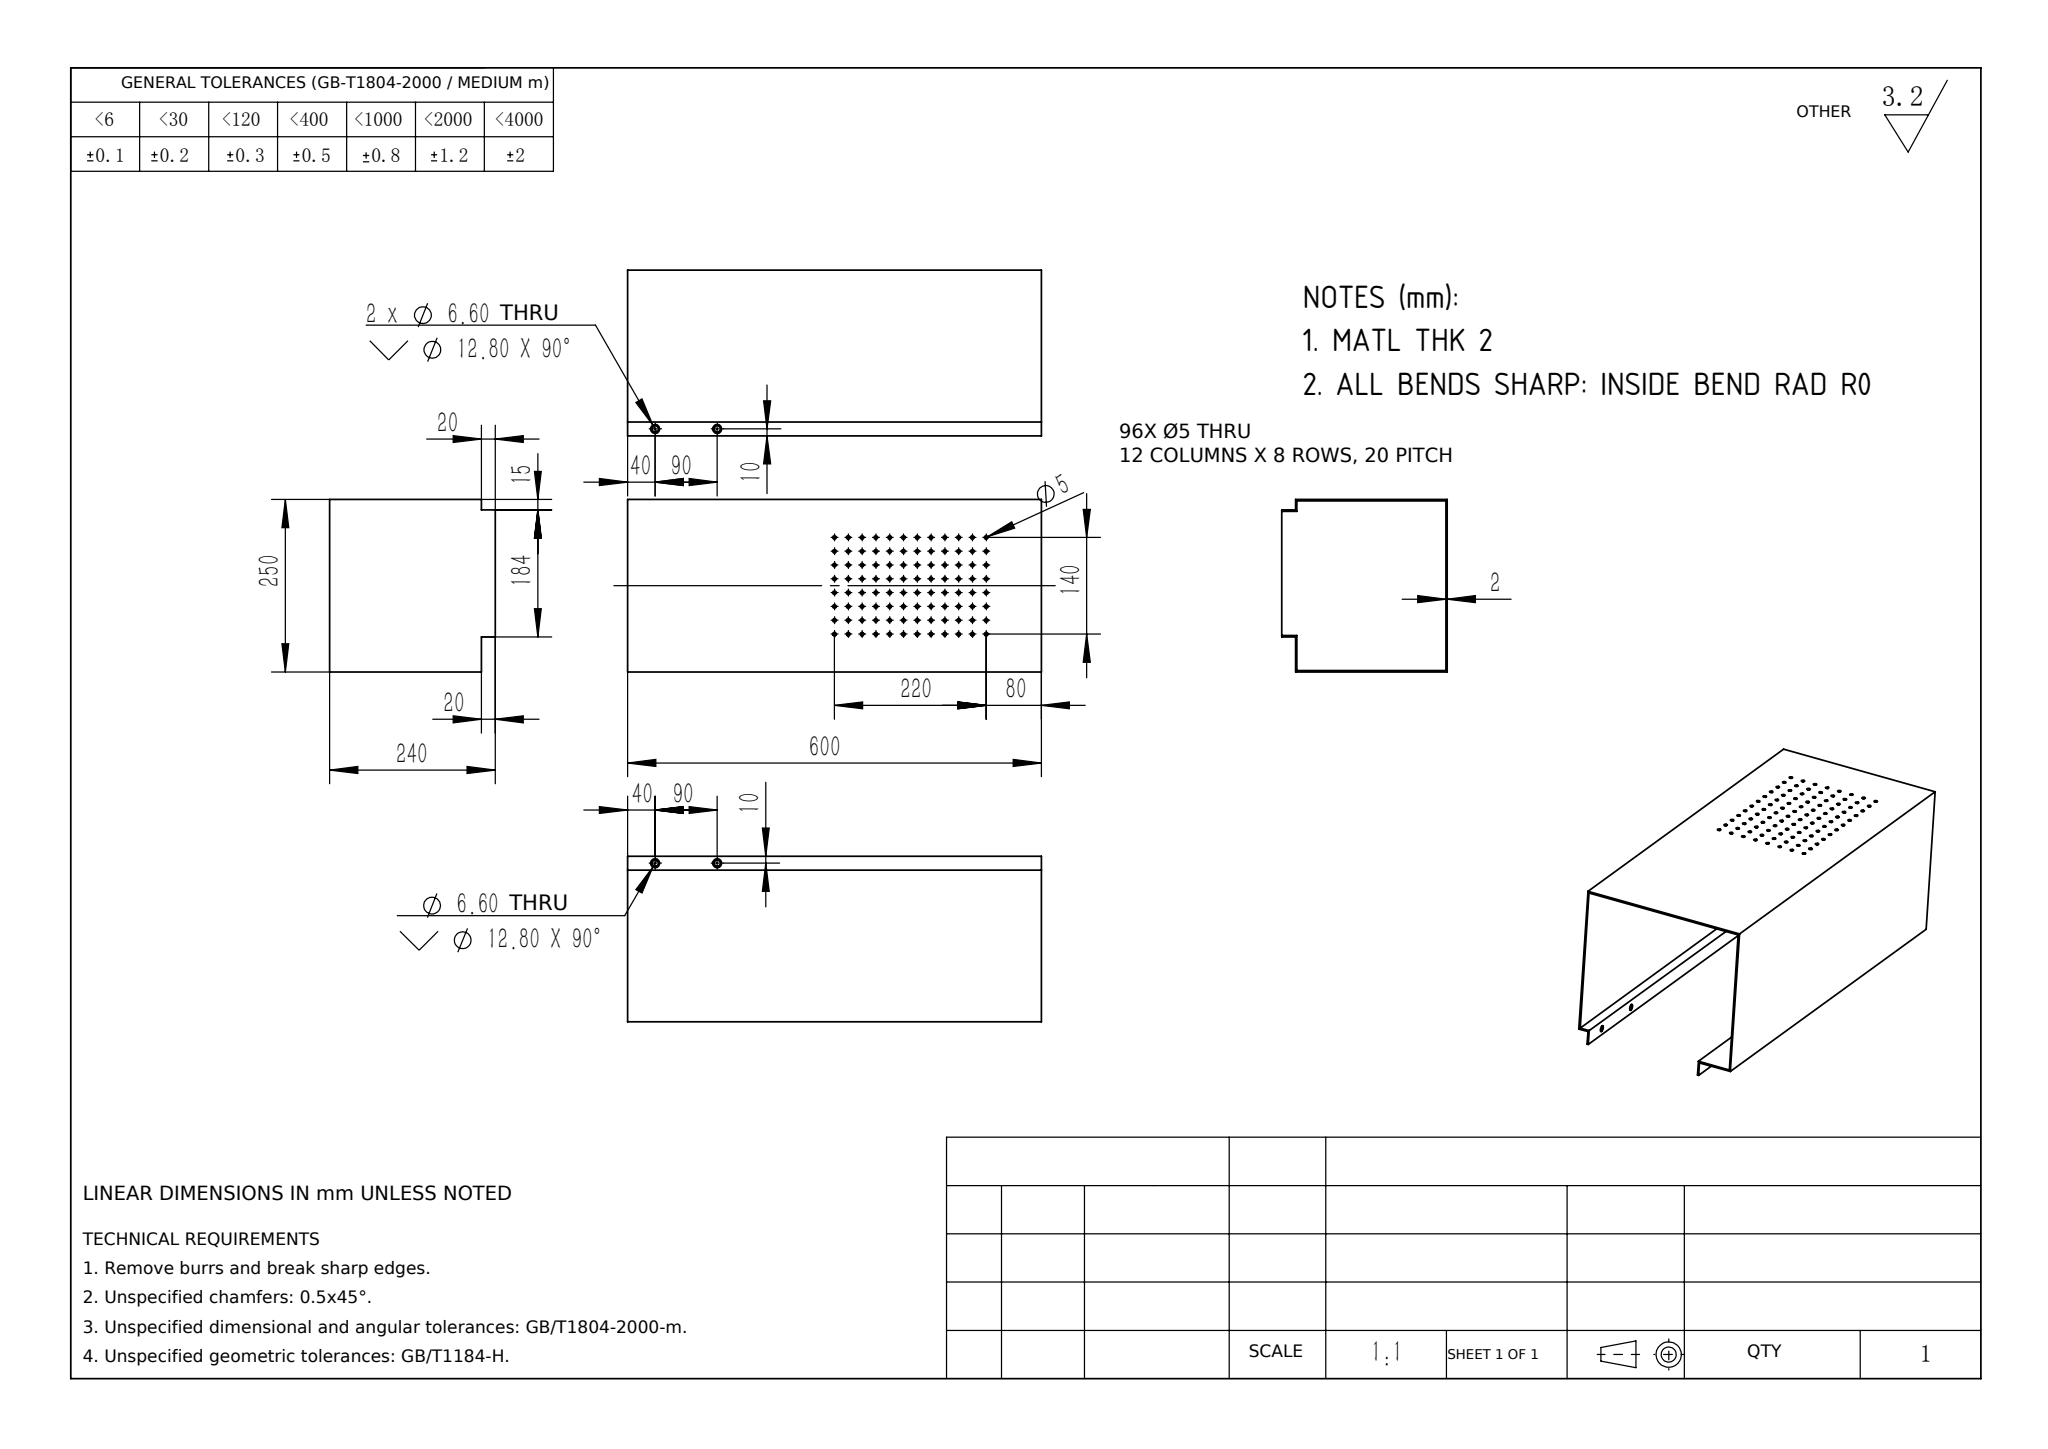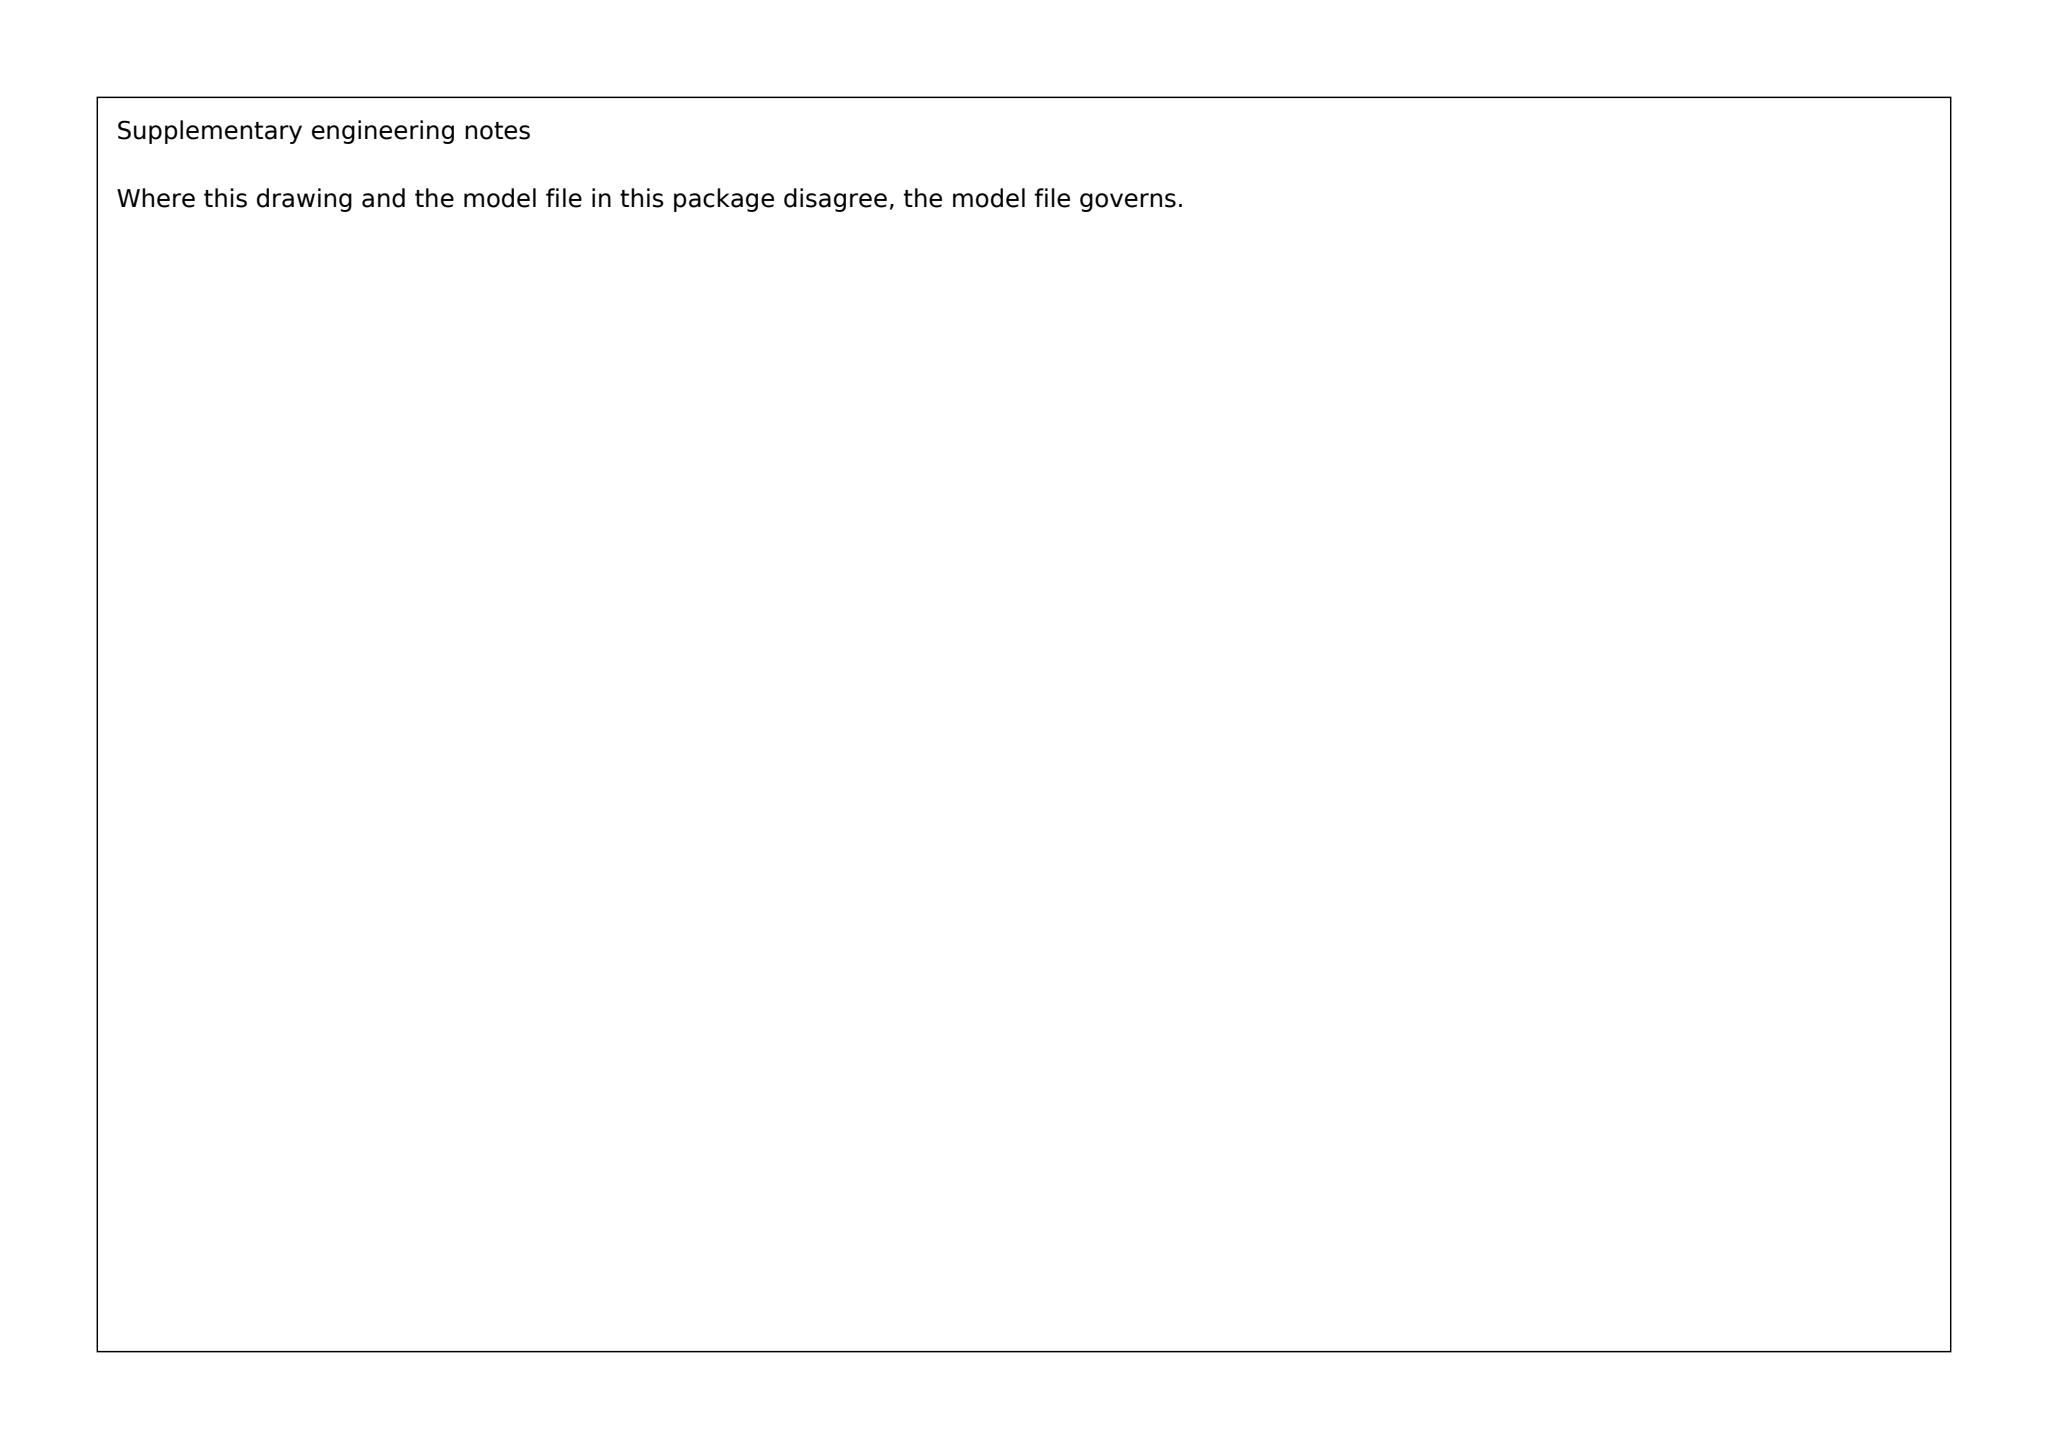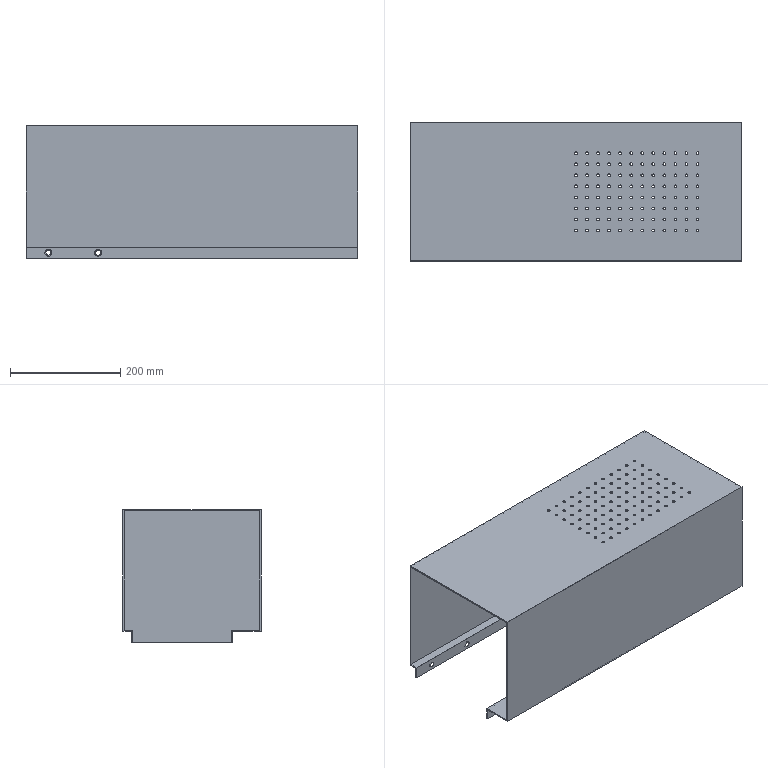Part | SolidWorks | mm | 1 solid | 218 faces | box 600 x 250 x 240 mm | volume 1060081 mm3 | cylinder 192 | plane 18 | cone 8 | commonest cylinder face diameters 5 x192
Drawing notes:
MATL THK 2 | from the solid: offset plane pairs y=0/2, y=248/250, z=20/22, z=238/240 show uniform 2 thk
ALL BENDS SHARP: INSIDE BEND RAD R0 | from the solid: fillet_radii list empty; no radii at bend plane pairs
build123d program:
from build123d import *

# Parameters (mm, degrees)
SKETCH1_W                                         = 600
SKETCH1_H                                         = 250
BOSS_EXTRUDE1_DEPTH                               = 240
SHELL1_T                                          = -2
SKETCH3_W                                         = 598
SKETCH3_H                                         = 2
CUT_EXTRUDE1_DEPTH                                = 22
SKETCH4_W                                         = 598
SKETCH4_H                                         = 17
BOSS_EXTRUDE2_DEPTH                               = 2
SKETCH5_W                                         = 598
SKETCH5_H                                         = 2
BOSS_EXTRUDE3_DEPTH                               = 20
SKETCH6_W                                         = 20
SKETCH6_H                                         = 15
CUT_EXTRUDE2_DEPTH                                = 657.376
SKETCH7_W                                         = 598
SKETCH7_H                                         = 2
CUT_EXTRUDE3_DEPTH                                = 22
SKETCH8_W                                         = 598
SKETCH8_H                                         = 53
BOSS_EXTRUDE4_DEPTH                               = 2
SKETCH9_W                                         = 598
SKETCH9_H                                         = 2
BOSS_EXTRUDE5_DEPTH                               = 20
SKETCH10_W                                        = 20
SKETCH10_H                                        = 51
CUT_EXTRUDE4_DEPTH                                = 657.376
HOLE_SIZE_ACCORDING_TO_HEXALOBULAR_RA_D           = 6.6
HOLE_SIZE_ACCORDING_TO_HEXALOBULAR_RA_CSINK_D     = 12.8
HOLE_SIZE_ACCORDING_TO_HEXALOBULAR_RA_CSINK_ANGLE = 90
HOLE_SIZE_ACCORDING_TO_HEXALOBULA_2_D             = 6.6
HOLE_SIZE_ACCORDING_TO_HEXALOBULA_2_CSINK_D       = 12.8
HOLE_SIZE_ACCORDING_TO_HEXALOBULA_2_CSINK_ANGLE   = 90
SKETCH15_R                                        = 2.5
CUT_EXTRUDE5_DEPTH                                = 2


with BuildPart() as part:
    # Sketch1 → Boss-Extrude1 (new body)
    with BuildSketch(Plane.XY):
        Rectangle(SKETCH1_W, SKETCH1_H)
    extrude(amount=BOSS_EXTRUDE1_DEPTH)

    # Shell1
    shell1_openings = [part.faces().sort_by_distance(p)[0] for p in [
        (0, 0, 0),
        (-300, 0, 120),
    ]]
    offset(amount=SHELL1_T, openings=shell1_openings, kind=Kind.INTERSECTION)

    # Sketch3 → Cut-Extrude1 (cut)
    with BuildSketch(Plane(origin=(0, 0, 0), x_dir=(-1, 0, 0), z_dir=(0, 0, -1))):
        with Locations((1, 124)):
            Rectangle(SKETCH3_W, SKETCH3_H)
    extrude(amount=-CUT_EXTRUDE1_DEPTH, mode=Mode.SUBTRACT)

    # Sketch4 → Boss-Extrude2 (add)
    with BuildSketch(Plane(origin=(0, 0, 22), x_dir=(-1, 0, 0), z_dir=(0, 0, -1))):
        with Locations((1, 116.5)):
            Rectangle(SKETCH4_W, SKETCH4_H)
    extrude(amount=BOSS_EXTRUDE2_DEPTH)

    # Sketch5 → Boss-Extrude3 (add)
    with BuildSketch(Plane(origin=(0, 0, 20), x_dir=(-1, 0, 0), z_dir=(0, 0, -1))):
        with Locations((1, 109)):
            Rectangle(SKETCH5_W, SKETCH5_H)
    extrude(amount=BOSS_EXTRUDE3_DEPTH)

    # Sketch6 → Cut-Extrude2 (cut, through all)
    with BuildSketch(Plane.ZY.offset(-298)):
        with Locations((10, 117.5)):
            Rectangle(SKETCH6_W, SKETCH6_H)
    extrude(amount=-CUT_EXTRUDE2_DEPTH, mode=Mode.SUBTRACT)

    # Sketch7 → Cut-Extrude3 (cut)
    with BuildSketch(Plane(origin=(0, 0, 0), x_dir=(-1, 0, 0), z_dir=(0, 0, -1))):
        with Locations((1, -124)):
            Rectangle(SKETCH7_W, SKETCH7_H)
    extrude(amount=-CUT_EXTRUDE3_DEPTH, mode=Mode.SUBTRACT)

    # Sketch8 → Boss-Extrude4 (add)
    with BuildSketch(Plane(origin=(0, 0, 22), x_dir=(-1, 0, 0), z_dir=(0, 0, -1))):
        with Locations((1, -98.5)):
            Rectangle(SKETCH8_W, SKETCH8_H)
    extrude(amount=BOSS_EXTRUDE4_DEPTH)

    # Sketch9 → Boss-Extrude5 (add)
    with BuildSketch(Plane(origin=(0, 0, 20), x_dir=(-1, 0, 0), z_dir=(0, 0, -1))):
        with Locations((1, -73)):
            Rectangle(SKETCH9_W, SKETCH9_H)
    extrude(amount=BOSS_EXTRUDE5_DEPTH)

    # Sketch10 → Cut-Extrude4 (cut, through all)
    with BuildSketch(Plane.ZY.offset(-298)):
        with Locations((10, -99.5)):
            Rectangle(SKETCH10_W, SKETCH10_H)
    extrude(amount=-CUT_EXTRUDE4_DEPTH, mode=Mode.SUBTRACT)

    # Hole Size _ according to_ Hexalobular Ra (through all)
    with Locations(Plane(origin=(0, 110, 0), x_dir=(1, 0, 0), z_dir=(0, 1, 0))):
        with Locations((-260, -10), (-170, -10)):
            CounterSinkHole(HOLE_SIZE_ACCORDING_TO_HEXALOBULAR_RA_D / 2, HOLE_SIZE_ACCORDING_TO_HEXALOBULAR_RA_CSINK_D / 2, counter_sink_angle=HOLE_SIZE_ACCORDING_TO_HEXALOBULAR_RA_CSINK_ANGLE)

    # Hole Size _ according to_ Hexalobula 2 (through all)
    with Locations(Plane(origin=(0, -74, 0), x_dir=(-1, 0, 0), z_dir=(0, -1, 0))):
        with Locations((260, -10), (170, -10)):
            CounterSinkHole(HOLE_SIZE_ACCORDING_TO_HEXALOBULA_2_D / 2, HOLE_SIZE_ACCORDING_TO_HEXALOBULA_2_CSINK_D / 2, counter_sink_angle=HOLE_SIZE_ACCORDING_TO_HEXALOBULA_2_CSINK_ANGLE)

    # Sketch15 → Cut-Extrude5 (cut)
    with BuildSketch(Plane.XY.offset(240)):
        with Locations((0, 70)):
            Circle(SKETCH15_R)
        with Locations((20, 70)):
            Circle(SKETCH15_R)
        with Locations((40, 70)):
            Circle(SKETCH15_R)
        with Locations((60, 70)):
            Circle(SKETCH15_R)
        with Locations((80, 70)):
            Circle(SKETCH15_R)
        with Locations((100, 70)):
            Circle(SKETCH15_R)
        with Locations((120, 70)):
            Circle(SKETCH15_R)
        with Locations((140, 70)):
            Circle(SKETCH15_R)
        with Locations((160, 70)):
            Circle(SKETCH15_R)
        with Locations((180, 70)):
            Circle(SKETCH15_R)
        with Locations((200, 70)):
            Circle(SKETCH15_R)
        with Locations((220, 70)):
            Circle(SKETCH15_R)
        with Locations((20, 50)):
            Circle(SKETCH15_R)
        with Locations((40, 50)):
            Circle(SKETCH15_R)
        with Locations((60, 50)):
            Circle(SKETCH15_R)
        with Locations((80, 50)):
            Circle(SKETCH15_R)
        with Locations((100, 50)):
            Circle(SKETCH15_R)
        with Locations((120, 50)):
            Circle(SKETCH15_R)
        with Locations((140, 50)):
            Circle(SKETCH15_R)
        with Locations((160, 50)):
            Circle(SKETCH15_R)
        with Locations((180, 50)):
            Circle(SKETCH15_R)
        with Locations((200, 50)):
            Circle(SKETCH15_R)
        with Locations((220, 50)):
            Circle(SKETCH15_R)
        with Locations((20, 30)):
            Circle(SKETCH15_R)
        with Locations((40, 30)):
            Circle(SKETCH15_R)
        with Locations((60, 30)):
            Circle(SKETCH15_R)
        with Locations((80, 30)):
            Circle(SKETCH15_R)
        with Locations((100, 30)):
            Circle(SKETCH15_R)
        with Locations((120, 30)):
            Circle(SKETCH15_R)
        with Locations((140, 30)):
            Circle(SKETCH15_R)
        with Locations((160, 30)):
            Circle(SKETCH15_R)
        with Locations((180, 30)):
            Circle(SKETCH15_R)
        with Locations((200, 30)):
            Circle(SKETCH15_R)
        with Locations((220, 30)):
            Circle(SKETCH15_R)
        with Locations((20, 10)):
            Circle(SKETCH15_R)
        with Locations((40, 10)):
            Circle(SKETCH15_R)
        with Locations((60, 10)):
            Circle(SKETCH15_R)
        with Locations((80, 10)):
            Circle(SKETCH15_R)
        with Locations((100, 10)):
            Circle(SKETCH15_R)
        with Locations((120, 10)):
            Circle(SKETCH15_R)
        with Locations((140, 10)):
            Circle(SKETCH15_R)
        with Locations((160, 10)):
            Circle(SKETCH15_R)
        with Locations((180, 10)):
            Circle(SKETCH15_R)
        with Locations((200, 10)):
            Circle(SKETCH15_R)
        with Locations((220, 10)):
            Circle(SKETCH15_R)
        with Locations((20, -10)):
            Circle(SKETCH15_R)
        with Locations((40, -10)):
            Circle(SKETCH15_R)
        with Locations((60, -10)):
            Circle(SKETCH15_R)
        with Locations((80, -10)):
            Circle(SKETCH15_R)
        with Locations((100, -10)):
            Circle(SKETCH15_R)
        with Locations((120, -10)):
            Circle(SKETCH15_R)
        with Locations((140, -10)):
            Circle(SKETCH15_R)
        with Locations((160, -10)):
            Circle(SKETCH15_R)
        with Locations((180, -10)):
            Circle(SKETCH15_R)
        with Locations((200, -10)):
            Circle(SKETCH15_R)
        with Locations((220, -10)):
            Circle(SKETCH15_R)
        with Locations((20, -30)):
            Circle(SKETCH15_R)
        with Locations((40, -30)):
            Circle(SKETCH15_R)
        with Locations((60, -30)):
            Circle(SKETCH15_R)
        with Locations((80, -30)):
            Circle(SKETCH15_R)
        with Locations((100, -30)):
            Circle(SKETCH15_R)
        with Locations((120, -30)):
            Circle(SKETCH15_R)
        with Locations((140, -30)):
            Circle(SKETCH15_R)
        with Locations((160, -30)):
            Circle(SKETCH15_R)
        with Locations((180, -30)):
            Circle(SKETCH15_R)
        with Locations((200, -30)):
            Circle(SKETCH15_R)
        with Locations((220, -30)):
            Circle(SKETCH15_R)
        with Locations((20, -50)):
            Circle(SKETCH15_R)
        with Locations((40, -50)):
            Circle(SKETCH15_R)
        with Locations((60, -50)):
            Circle(SKETCH15_R)
        with Locations((80, -50)):
            Circle(SKETCH15_R)
        with Locations((100, -50)):
            Circle(SKETCH15_R)
        with Locations((120, -50)):
            Circle(SKETCH15_R)
        with Locations((140, -50)):
            Circle(SKETCH15_R)
        with Locations((160, -50)):
            Circle(SKETCH15_R)
        with Locations((180, -50)):
            Circle(SKETCH15_R)
        with Locations((200, -50)):
            Circle(SKETCH15_R)
        with Locations((220, -50)):
            Circle(SKETCH15_R)
        with Locations((20, -70)):
            Circle(SKETCH15_R)
        with Locations((40, -70)):
            Circle(SKETCH15_R)
        with Locations((60, -70)):
            Circle(SKETCH15_R)
        with Locations((80, -70)):
            Circle(SKETCH15_R)
        with Locations((100, -70)):
            Circle(SKETCH15_R)
        with Locations((120, -70)):
            Circle(SKETCH15_R)
        with Locations((140, -70)):
            Circle(SKETCH15_R)
        with Locations((160, -70)):
            Circle(SKETCH15_R)
        with Locations((180, -70)):
            Circle(SKETCH15_R)
        with Locations((200, -70)):
            Circle(SKETCH15_R)
        with Locations((220, -70)):
            Circle(SKETCH15_R)
        with Locations((0, 50)):
            Circle(SKETCH15_R)
        with Locations((0, 30)):
            Circle(SKETCH15_R)
        with Locations((0, 10)):
            Circle(SKETCH15_R)
        with Locations((0, -10)):
            Circle(SKETCH15_R)
        with Locations((0, -30)):
            Circle(SKETCH15_R)
        with Locations((0, -50)):
            Circle(SKETCH15_R)
        with Locations((0, -70)):
            Circle(SKETCH15_R)
    extrude(amount=-CUT_EXTRUDE5_DEPTH, mode=Mode.SUBTRACT)


solid = part.part